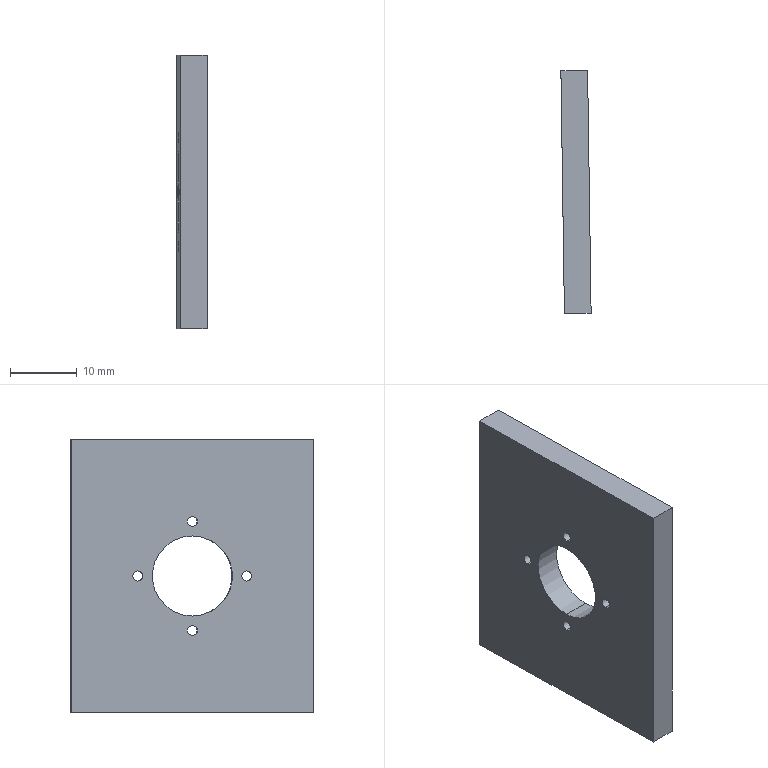Component | SolidWorks | MiddleBaffle-1 | 1 solid | 16 faces | box 4.53 x 36.32 x 41 mm | volume 5472 mm3 | cylinder 10 | plane 6 | commonest cylinder face diameters 1.5 x8 12 x2
build123d program:
from build123d import *

# Parameters (mm, degrees)
SKETCH1_2_W                 = 41
SKETCH1_2_H                 = 36.324
BOSS_EXTRUDE1_DEPTH         = 4
CUT_EXTRUDE1_DEPTH          = 56.157
CUT_EXTRUDE1_DEPTH_BACK     = 56.157
SKETCH2_R                   = 6
SKETCH3_R                   = 0.75
CUT_EXTRUDE2_DEPTH          = 56.157
CIRPATTERN1_COUNT           = 4
BOTTOM_SEAT_TRIM_DEPTH      = 56.157
BOTTOM_SEAT_TRIM_DEPTH_BACK = 56.157


with BuildPart() as part:
    # Sketch1_2 → Boss-Extrude1 (new body)
    with BuildSketch(Plane.XY):
        with Locations((1, 32.475)):
            Rectangle(SKETCH1_2_W, SKETCH1_2_H)
    extrude(amount=BOSS_EXTRUDE1_DEPTH)

    # Sketch2 → Cut-Extrude1 (cut, two sides: drawn at the far end of the back side and taken through both)
    with BuildSketch(Plane.XY.offset(4).offset(-CUT_EXTRUDE1_DEPTH_BACK)):
        with Locations((1, 32.475)):
            Circle(SKETCH2_R)
    extrude(amount=CUT_EXTRUDE1_DEPTH + CUT_EXTRUDE1_DEPTH_BACK, mode=Mode.SUBTRACT)

    # Sketch3 → Cut-Extrude2 (cut, symmetric)
    with BuildSketch(Plane.XY.offset(4)):
        with Locations((1, 40.63)):
            Circle(SKETCH3_R)
    cut_extrude2 = extrude(amount=CUT_EXTRUDE2_DEPTH, both=True, mode=Mode.SUBTRACT)

    # CirPattern1: Cut-Extrude2 ×4 about axis
    cirpattern1_axis = Axis((1, 32.475, 0), (0, 0, 1))
    for i in range(1, CIRPATTERN1_COUNT):
        add(cut_extrude2.rotate(cirpattern1_axis, i * 360 / CIRPATTERN1_COUNT), mode=Mode.SUBTRACT)

    # Sketch1 → Bottom seat trim (cut, two sides: drawn at the far end of the back side and taken through both)
    with BuildSketch(Plane(origin=(0, 0, 0), x_dir=(0, 0, -1), z_dir=(1, 0, 0)).offset(-BOTTOM_SEAT_TRIM_DEPTH_BACK)):
        Polygon((0.5, 14.305), (-4.5, 14.378), (-4.5, 13.9), (0.5, 13.9), align=None)
    extrude(amount=BOTTOM_SEAT_TRIM_DEPTH + BOTTOM_SEAT_TRIM_DEPTH_BACK, mode=Mode.SUBTRACT)


solid = part.part

# Placed as in the assembly
solid = solid.moved(Location((90.898, 1.581, 0), (90, -89.169, 90)))
STEP:
#1=COLOUR_RGB('',0.7922,0.8196,0.9333);
#2=FILL_AREA_STYLE_COLOUR('',#1);
#3=FILL_AREA_STYLE('',(#2));
#4=SURFACE_STYLE_FILL_AREA(#3);
#5=SURFACE_SIDE_STYLE('',(#4));
#6=SURFACE_STYLE_USAGE(.BOTH.,#5);
#7=PRESENTATION_STYLE_ASSIGNMENT((#6));
#8=CARTESIAN_POINT('',(3.56,1.341,-0.3112));
#9=VERTEX_POINT('',#8);
#10=CARTESIAN_POINT('',(3.56,1.341,-0.2522));
#11=VERTEX_POINT('',#10);
#12=CARTESIAN_POINT('',(3.56,1.341,-0.2817));
#13=DIRECTION('',(-0.9999,-0.0145,0.));
#14=DIRECTION('',(-0.0145,0.9999,-0.));
#15=AXIS2_PLACEMENT_3D('',#12,#13,#14);
#16=CIRCLE('',#15,0.02953);
#17=EDGE_CURVE('',#9,#11,#16,.T.);
#18=ORIENTED_EDGE('',*,*,#17,.F.);
#19=CARTESIAN_POINT('',(3.403,1.338,-0.3112));
#20=VERTEX_POINT('',#19);
#21=CARTESIAN_POINT('',(3.56,1.341,-0.3112));
#22=DIRECTION('',(-0.9999,-0.0145,0.));
#23=VECTOR('',#22,39.37);
#24=LINE('',#21,#23);
#25=EDGE_CURVE('',#9,#20,#24,.T.);
#26=ORIENTED_EDGE('',*,*,#25,.T.);
#27=CARTESIAN_POINT('',(3.403,1.338,-0.2522));
#28=VERTEX_POINT('',#27);
#29=CARTESIAN_POINT('',(3.403,1.338,-0.2817));
#30=DIRECTION('',(-0.9999,-0.0145,0.));
#31=DIRECTION('',(0.,0.,1.));
#32=AXIS2_PLACEMENT_3D('',#29,#30,#31);
#33=CIRCLE('',#32,0.02953);
#34=EDGE_CURVE('',#20,#28,#33,.T.);
#35=ORIENTED_EDGE('',*,*,#34,.T.);
#36=CARTESIAN_POINT('',(3.56,1.341,-0.2522));
#37=DIRECTION('',(-0.9999,-0.0145,0.));
#38=VECTOR('',#37,39.37);
#39=LINE('',#36,#38);
#40=EDGE_CURVE('',#11,#28,#39,.T.);
#41=ORIENTED_EDGE('',*,*,#40,.F.);
#42=EDGE_LOOP('',(#18,#26,#35,#41));
#43=FACE_OUTER_BOUND('',#42,.T.);
#44=CARTESIAN_POINT('',(3.56,1.341,-0.2817));
#45=DIRECTION('',(-0.9999,-0.0145,0.));
#46=DIRECTION('',(0.,0.,1.));
#47=AXIS2_PLACEMENT_3D('',#44,#45,#46);
#48=CYLINDRICAL_SURFACE('',#47,0.02953);
#49=ADVANCED_FACE('',(#43),#48,.F.);
#50=CARTESIAN_POINT('',(3.565,1.02,0.009843));
#51=VERTEX_POINT('',#50);
#52=CARTESIAN_POINT('',(3.565,1.02,0.0689));
#53=VERTEX_POINT('',#52);
#54=CARTESIAN_POINT('',(3.565,1.02,0.03937));
#55=DIRECTION('',(-0.9999,-0.0145,0.));
#56=DIRECTION('',(0.,0.,-1.));
#57=AXIS2_PLACEMENT_3D('',#54,#55,#56);
#58=CIRCLE('',#57,0.02953);
#59=EDGE_CURVE('',#51,#53,#58,.T.);
#60=ORIENTED_EDGE('',*,*,#59,.F.);
#61=CARTESIAN_POINT('',(3.407,1.017,0.009843));
#62=VERTEX_POINT('',#61);
#63=CARTESIAN_POINT('',(3.565,1.02,0.009843));
#64=DIRECTION('',(-0.9999,-0.0145,0.));
#65=VECTOR('',#64,39.37);
#66=LINE('',#63,#65);
#67=EDGE_CURVE('',#51,#62,#66,.T.);
#68=ORIENTED_EDGE('',*,*,#67,.T.);
#69=CARTESIAN_POINT('',(3.407,1.017,0.0689));
#70=VERTEX_POINT('',#69);
#71=CARTESIAN_POINT('',(3.407,1.017,0.03937));
#72=DIRECTION('',(-0.9999,-0.0145,0.));
#73=DIRECTION('',(0.,0.,1.));
#74=AXIS2_PLACEMENT_3D('',#71,#72,#73);
#75=CIRCLE('',#74,0.02953);
#76=EDGE_CURVE('',#62,#70,#75,.T.);
#77=ORIENTED_EDGE('',*,*,#76,.T.);
#78=CARTESIAN_POINT('',(3.565,1.02,0.0689));
#79=DIRECTION('',(-0.9999,-0.0145,0.));
#80=VECTOR('',#79,39.37);
#81=LINE('',#78,#80);
#82=EDGE_CURVE('',#53,#70,#81,.T.);
#83=ORIENTED_EDGE('',*,*,#82,.F.);
#84=EDGE_LOOP('',(#60,#68,#77,#83));
#85=FACE_OUTER_BOUND('',#84,.T.);
#86=CARTESIAN_POINT('',(3.565,1.02,0.03937));
#87=DIRECTION('',(-0.9999,-0.0145,0.));
#88=DIRECTION('',(0.,0.,1.));
#89=AXIS2_PLACEMENT_3D('',#86,#87,#88);
#90=CYLINDRICAL_SURFACE('',#89,0.02953);
#91=ADVANCED_FACE('',(#85),#90,.F.);
#92=CARTESIAN_POINT('',(3.56,1.341,0.3309));
#93=VERTEX_POINT('',#92);
#94=CARTESIAN_POINT('',(3.56,1.341,0.39));
#95=VERTEX_POINT('',#94);
#96=CARTESIAN_POINT('',(3.56,1.341,0.3604));
#97=DIRECTION('',(-0.9999,-0.0145,0.));
#98=DIRECTION('',(0.0145,-0.9999,0.));
#99=AXIS2_PLACEMENT_3D('',#96,#97,#98);
#100=CIRCLE('',#99,0.02953);
#101=EDGE_CURVE('',#93,#95,#100,.T.);
#102=ORIENTED_EDGE('',*,*,#101,.F.);
#103=CARTESIAN_POINT('',(3.403,1.338,0.3309));
#104=VERTEX_POINT('',#103);
#105=CARTESIAN_POINT('',(3.56,1.341,0.3309));
#106=DIRECTION('',(-0.9999,-0.0145,0.));
#107=VECTOR('',#106,39.37);
#108=LINE('',#105,#107);
#109=EDGE_CURVE('',#93,#104,#108,.T.);
#110=ORIENTED_EDGE('',*,*,#109,.T.);
#111=CARTESIAN_POINT('',(3.403,1.338,0.39));
#112=VERTEX_POINT('',#111);
#113=CARTESIAN_POINT('',(3.403,1.338,0.3604));
#114=DIRECTION('',(-0.9999,-0.0145,0.));
#115=DIRECTION('',(0.,0.,1.));
#116=AXIS2_PLACEMENT_3D('',#113,#114,#115);
#117=CIRCLE('',#116,0.02953);
#118=EDGE_CURVE('',#104,#112,#117,.T.);
#119=ORIENTED_EDGE('',*,*,#118,.T.);
#120=CARTESIAN_POINT('',(3.56,1.341,0.39));
#121=DIRECTION('',(-0.9999,-0.0145,0.));
#122=VECTOR('',#121,39.37);
#123=LINE('',#120,#122);
#124=EDGE_CURVE('',#95,#112,#123,.T.);
#125=ORIENTED_EDGE('',*,*,#124,.F.);
#126=EDGE_LOOP('',(#102,#110,#119,#125));
#127=FACE_OUTER_BOUND('',#126,.T.);
#128=CARTESIAN_POINT('',(3.56,1.341,0.3604));
#129=DIRECTION('',(-0.9999,-0.0145,0.));
#130=DIRECTION('',(0.,0.,1.));
#131=AXIS2_PLACEMENT_3D('',#128,#129,#130);
#132=CYLINDRICAL_SURFACE('',#131,0.02953);
#133=ADVANCED_FACE('',(#127),#132,.F.);
#134=CARTESIAN_POINT('',(3.555,1.662,0.009843));
#135=VERTEX_POINT('',#134);
#136=CARTESIAN_POINT('',(3.555,1.662,0.0689));
#137=VERTEX_POINT('',#136);
#138=CARTESIAN_POINT('',(3.555,1.662,0.03937));
#139=DIRECTION('',(-0.9999,-0.0145,0.));
#140=DIRECTION('',(0.,0.,1.));
#141=AXIS2_PLACEMENT_3D('',#138,#139,#140);
#142=CIRCLE('',#141,0.02953);
#143=EDGE_CURVE('',#135,#137,#142,.T.);
#144=ORIENTED_EDGE('',*,*,#143,.F.);
#145=CARTESIAN_POINT('',(3.398,1.659,0.009843));
#146=VERTEX_POINT('',#145);
#147=CARTESIAN_POINT('',(3.555,1.662,0.009843));
#148=DIRECTION('',(-0.9999,-0.0145,0.));
#149=VECTOR('',#148,39.37);
#150=LINE('',#147,#149);
#151=EDGE_CURVE('',#135,#146,#150,.T.);
#152=ORIENTED_EDGE('',*,*,#151,.T.);
#153=CARTESIAN_POINT('',(3.398,1.659,0.0689));
#154=VERTEX_POINT('',#153);
#155=CARTESIAN_POINT('',(3.398,1.659,0.03937));
#156=DIRECTION('',(-0.9999,-0.0145,0.));
#157=DIRECTION('',(0.,0.,1.));
#158=AXIS2_PLACEMENT_3D('',#155,#156,#157);
#159=CIRCLE('',#158,0.02953);
#160=EDGE_CURVE('',#146,#154,#159,.T.);
#161=ORIENTED_EDGE('',*,*,#160,.T.);
#162=CARTESIAN_POINT('',(3.555,1.662,0.0689));
#163=DIRECTION('',(-0.9999,-0.0145,0.));
#164=VECTOR('',#163,39.37);
#165=LINE('',#162,#164);
#166=EDGE_CURVE('',#137,#154,#165,.T.);
#167=ORIENTED_EDGE('',*,*,#166,.F.);
#168=EDGE_LOOP('',(#144,#152,#161,#167));
#169=FACE_OUTER_BOUND('',#168,.T.);
#170=CARTESIAN_POINT('',(3.555,1.662,0.03937));
#171=DIRECTION('',(-0.9999,-0.0145,0.));
#172=DIRECTION('',(0.,0.,1.));
#173=AXIS2_PLACEMENT_3D('',#170,#171,#172);
#174=CYLINDRICAL_SURFACE('',#173,0.02953);
#175=ADVANCED_FACE('',(#169),#174,.F.);
#176=CARTESIAN_POINT('',(3.56,1.341,-0.1969));
#177=VERTEX_POINT('',#176);
#178=CARTESIAN_POINT('',(3.56,1.341,0.2756));
#179=VERTEX_POINT('',#178);
#180=CARTESIAN_POINT('',(3.56,1.341,0.03937));
#181=DIRECTION('',(-0.9999,-0.0145,0.));
#182=DIRECTION('',(0.,0.,1.));
#183=AXIS2_PLACEMENT_3D('',#180,#181,#182);
#184=CIRCLE('',#183,0.2362);
#185=EDGE_CURVE('',#177,#179,#184,.T.);
#186=ORIENTED_EDGE('',*,*,#185,.F.);
#187=CARTESIAN_POINT('',(3.403,1.338,-0.1969));
#188=VERTEX_POINT('',#187);
#189=CARTESIAN_POINT('',(3.56,1.341,-0.1969));
#190=DIRECTION('',(-0.9999,-0.0145,0.));
#191=VECTOR('',#190,39.37);
#192=LINE('',#189,#191);
#193=EDGE_CURVE('',#177,#188,#192,.T.);
#194=ORIENTED_EDGE('',*,*,#193,.T.);
#195=CARTESIAN_POINT('',(3.403,1.338,0.2756));
#196=VERTEX_POINT('',#195);
#197=CARTESIAN_POINT('',(3.403,1.338,0.03937));
#198=DIRECTION('',(-0.9999,-0.0145,0.));
#199=DIRECTION('',(0.,0.,1.));
#200=AXIS2_PLACEMENT_3D('',#197,#198,#199);
#201=CIRCLE('',#200,0.2362);
#202=EDGE_CURVE('',#188,#196,#201,.T.);
#203=ORIENTED_EDGE('',*,*,#202,.T.);
#204=CARTESIAN_POINT('',(3.56,1.341,0.2756));
#205=DIRECTION('',(-0.9999,-0.0145,0.));
#206=VECTOR('',#205,39.37);
#207=LINE('',#204,#206);
#208=EDGE_CURVE('',#179,#196,#207,.T.);
#209=ORIENTED_EDGE('',*,*,#208,.F.);
#210=EDGE_LOOP('',(#186,#194,#203,#209));
#211=FACE_OUTER_BOUND('',#210,.T.);
#212=CARTESIAN_POINT('',(3.56,1.341,0.03937));
#213=DIRECTION('',(-0.9999,-0.0145,0.));
#214=DIRECTION('',(0.,0.,1.));
#215=AXIS2_PLACEMENT_3D('',#212,#213,#214);
#216=CYLINDRICAL_SURFACE('',#215,0.2362);
#217=ADVANCED_FACE('',(#211),#216,.F.);
#218=CARTESIAN_POINT('',(3.57,0.6257,0.8465));
#219=VERTEX_POINT('',#218);
#220=CARTESIAN_POINT('',(3.413,0.6257,0.8465));
#221=VERTEX_POINT('',#220);
#222=CARTESIAN_POINT('',(3.59,0.6257,0.8465));
#223=DIRECTION('',(-1.,0.0000005,0.));
#224=VECTOR('',#223,39.37);
#225=LINE('',#222,#224);
#226=EDGE_CURVE('',#219,#221,#225,.T.);
#227=ORIENTED_EDGE('',*,*,#226,.F.);
#228=CARTESIAN_POINT('',(3.55,2.056,0.8465));
#229=VERTEX_POINT('',#228);
#230=CARTESIAN_POINT('',(3.55,2.056,0.8465));
#231=DIRECTION('',(-0.0145,0.9999,0.));
#232=VECTOR('',#231,39.37);
#233=LINE('',#230,#232);
#234=EDGE_CURVE('',#219,#229,#233,.T.);
#235=ORIENTED_EDGE('',*,*,#234,.T.);
#236=CARTESIAN_POINT('',(3.392,2.053,0.8465));
#237=VERTEX_POINT('',#236);
#238=CARTESIAN_POINT('',(3.392,2.053,0.8465));
#239=DIRECTION('',(0.9999,0.0145,0.));
#240=VECTOR('',#239,39.37);
#241=LINE('',#238,#240);
#242=EDGE_CURVE('',#237,#229,#241,.T.);
#243=ORIENTED_EDGE('',*,*,#242,.F.);
#244=CARTESIAN_POINT('',(3.392,2.053,0.8465));
#245=DIRECTION('',(-0.0145,0.9999,0.));
#246=VECTOR('',#245,39.37);
#247=LINE('',#244,#246);
#248=EDGE_CURVE('',#221,#237,#247,.T.);
#249=ORIENTED_EDGE('',*,*,#248,.F.);
#250=EDGE_LOOP('',(#227,#235,#243,#249));
#251=FACE_OUTER_BOUND('',#250,.T.);
#252=CARTESIAN_POINT('',(3.392,2.053,0.8465));
#253=DIRECTION('',(0.,0.,-1.));
#254=DIRECTION('',(-0.9999,-0.0145,0.));
#255=AXIS2_PLACEMENT_3D('',#252,#253,#254);
#256=PLANE('',#255);
#257=ADVANCED_FACE('',(#251),#256,.F.);
#258=CARTESIAN_POINT('',(3.55,2.056,-0.7677));
#259=VERTEX_POINT('',#258);
#260=CARTESIAN_POINT('',(3.57,0.6257,-0.7677));
#261=VERTEX_POINT('',#260);
#262=CARTESIAN_POINT('',(3.55,2.056,-0.7677));
#263=DIRECTION('',(0.0145,-0.9999,0.));
#264=VECTOR('',#263,39.37);
#265=LINE('',#262,#264);
#266=EDGE_CURVE('',#259,#261,#265,.T.);
#267=ORIENTED_EDGE('',*,*,#266,.T.);
#268=CARTESIAN_POINT('',(3.413,0.6257,-0.7677));
#269=VERTEX_POINT('',#268);
#270=CARTESIAN_POINT('',(3.59,0.6257,-0.7677));
#271=DIRECTION('',(-1.,0.0000005,0.));
#272=VECTOR('',#271,39.37);
#273=LINE('',#270,#272);
#274=EDGE_CURVE('',#261,#269,#273,.T.);
#275=ORIENTED_EDGE('',*,*,#274,.T.);
#276=CARTESIAN_POINT('',(3.392,2.053,-0.7677));
#277=VERTEX_POINT('',#276);
#278=CARTESIAN_POINT('',(3.392,2.053,-0.7677));
#279=DIRECTION('',(0.0145,-0.9999,0.));
#280=VECTOR('',#279,39.37);
#281=LINE('',#278,#280);
#282=EDGE_CURVE('',#277,#269,#281,.T.);
#283=ORIENTED_EDGE('',*,*,#282,.F.);
#284=CARTESIAN_POINT('',(3.392,2.053,-0.7677));
#285=DIRECTION('',(0.9999,0.0145,0.));
#286=VECTOR('',#285,39.37);
#287=LINE('',#284,#286);
#288=EDGE_CURVE('',#277,#259,#287,.T.);
#289=ORIENTED_EDGE('',*,*,#288,.T.);
#290=EDGE_LOOP('',(#267,#275,#283,#289));
#291=FACE_OUTER_BOUND('',#290,.T.);
#292=CARTESIAN_POINT('',(3.392,2.053,-0.7677));
#293=DIRECTION('',(0.,0.,1.));
#294=DIRECTION('',(0.9999,0.0145,0.));
#295=AXIS2_PLACEMENT_3D('',#292,#293,#294);
#296=PLANE('',#295);
#297=ADVANCED_FACE('',(#291),#296,.F.);
#298=CARTESIAN_POINT('',(3.55,2.056,-0.7677));
#299=DIRECTION('',(0.,0.,-1.));
#300=VECTOR('',#299,39.37);
#301=LINE('',#298,#300);
#302=EDGE_CURVE('',#229,#259,#301,.T.);
#303=ORIENTED_EDGE('',*,*,#302,.T.);
#304=ORIENTED_EDGE('',*,*,#288,.F.);
#305=CARTESIAN_POINT('',(3.392,2.053,-0.7677));
#306=DIRECTION('',(0.,0.,-1.));
#307=VECTOR('',#306,39.37);
#308=LINE('',#305,#307);
#309=EDGE_CURVE('',#237,#277,#308,.T.);
#310=ORIENTED_EDGE('',*,*,#309,.F.);
#311=ORIENTED_EDGE('',*,*,#242,.T.);
#312=EDGE_LOOP('',(#303,#304,#310,#311));
#313=FACE_OUTER_BOUND('',#312,.T.);
#314=CARTESIAN_POINT('',(3.392,2.053,-0.7677));
#315=DIRECTION('',(0.0145,-0.9999,0.));
#316=DIRECTION('',(0.9999,0.0145,0.));
#317=AXIS2_PLACEMENT_3D('',#314,#315,#316);
#318=PLANE('',#317);
#319=ADVANCED_FACE('',(#313),#318,.F.);
#320=CARTESIAN_POINT('',(3.413,0.6257,0.));
#321=DIRECTION('',(0.,0.,-1.));
#322=VECTOR('',#321,39.37);
#323=LINE('',#320,#322);
#324=EDGE_CURVE('',#221,#269,#323,.T.);
#325=ORIENTED_EDGE('',*,*,#324,.F.);
#326=ORIENTED_EDGE('',*,*,#248,.T.);
#327=ORIENTED_EDGE('',*,*,#309,.T.);
#328=ORIENTED_EDGE('',*,*,#282,.T.);
#329=EDGE_LOOP('',(#325,#326,#327,#328));
#330=FACE_OUTER_BOUND('',#329,.T.);
#331=CARTESIAN_POINT('',(3.403,1.338,-0.2817));
#332=DIRECTION('',(-0.9999,-0.0145,0.));
#333=DIRECTION('',(0.,0.,1.));
#334=AXIS2_PLACEMENT_3D('',#331,#332,#333);
#335=CIRCLE('',#334,0.02953);
#336=EDGE_CURVE('',#28,#20,#335,.T.);
#337=ORIENTED_EDGE('',*,*,#336,.F.);
#338=ORIENTED_EDGE('',*,*,#34,.F.);
#339=EDGE_LOOP('',(#337,#338));
#340=FACE_BOUND('',#339,.T.);
#341=CARTESIAN_POINT('',(3.407,1.017,0.03937));
#342=DIRECTION('',(-0.9999,-0.0145,0.));
#343=DIRECTION('',(0.,0.,1.));
#344=AXIS2_PLACEMENT_3D('',#341,#342,#343);
#345=CIRCLE('',#344,0.02953);
#346=EDGE_CURVE('',#70,#62,#345,.T.);
#347=ORIENTED_EDGE('',*,*,#346,.F.);
#348=ORIENTED_EDGE('',*,*,#76,.F.);
#349=EDGE_LOOP('',(#347,#348));
#350=FACE_BOUND('',#349,.T.);
#351=CARTESIAN_POINT('',(3.403,1.338,0.3604));
#352=DIRECTION('',(-0.9999,-0.0145,0.));
#353=DIRECTION('',(0.,0.,1.));
#354=AXIS2_PLACEMENT_3D('',#351,#352,#353);
#355=CIRCLE('',#354,0.02953);
#356=EDGE_CURVE('',#112,#104,#355,.T.);
#357=ORIENTED_EDGE('',*,*,#356,.F.);
#358=ORIENTED_EDGE('',*,*,#118,.F.);
#359=EDGE_LOOP('',(#357,#358));
#360=FACE_BOUND('',#359,.T.);
#361=CARTESIAN_POINT('',(3.398,1.659,0.03937));
#362=DIRECTION('',(-0.9999,-0.0145,0.));
#363=DIRECTION('',(0.,0.,1.));
#364=AXIS2_PLACEMENT_3D('',#361,#362,#363);
#365=CIRCLE('',#364,0.02953);
#366=EDGE_CURVE('',#154,#146,#365,.T.);
#367=ORIENTED_EDGE('',*,*,#366,.F.);
#368=ORIENTED_EDGE('',*,*,#160,.F.);
#369=EDGE_LOOP('',(#367,#368));
#370=FACE_BOUND('',#369,.T.);
#371=CARTESIAN_POINT('',(3.403,1.338,0.03937));
#372=DIRECTION('',(-0.9999,-0.0145,0.));
#373=DIRECTION('',(0.,0.,1.));
#374=AXIS2_PLACEMENT_3D('',#371,#372,#373);
#375=CIRCLE('',#374,0.2362);
#376=EDGE_CURVE('',#196,#188,#375,.T.);
#377=ORIENTED_EDGE('',*,*,#376,.F.);
#378=ORIENTED_EDGE('',*,*,#202,.F.);
#379=EDGE_LOOP('',(#377,#378));
#380=FACE_BOUND('',#379,.T.);
#381=CARTESIAN_POINT('',(3.421,0.05994,0.));
#382=DIRECTION('',(-0.9999,-0.0145,0.));
#383=DIRECTION('',(0.,0.,1.));
#384=AXIS2_PLACEMENT_3D('',#381,#382,#383);
#385=PLANE('',#384);
#386=ADVANCED_FACE('',(#330,#340,#350,#360,#370,#380),#385,.T.);
#387=CARTESIAN_POINT('',(3.56,1.341,-0.2817));
#388=DIRECTION('',(-0.9999,-0.0145,0.));
#389=DIRECTION('',(-0.0145,0.9999,-0.));
#390=AXIS2_PLACEMENT_3D('',#387,#388,#389);
#391=CIRCLE('',#390,0.02953);
#392=EDGE_CURVE('',#11,#9,#391,.T.);
#393=ORIENTED_EDGE('',*,*,#392,.T.);
#394=ORIENTED_EDGE('',*,*,#17,.T.);
#395=EDGE_LOOP('',(#393,#394));
#396=FACE_BOUND('',#395,.T.);
#397=CARTESIAN_POINT('',(3.565,1.02,0.03937));
#398=DIRECTION('',(-0.9999,-0.0145,0.));
#399=DIRECTION('',(0.,0.,-1.));
#400=AXIS2_PLACEMENT_3D('',#397,#398,#399);
#401=CIRCLE('',#400,0.02953);
#402=EDGE_CURVE('',#53,#51,#401,.T.);
#403=ORIENTED_EDGE('',*,*,#402,.T.);
#404=ORIENTED_EDGE('',*,*,#59,.T.);
#405=EDGE_LOOP('',(#403,#404));
#406=FACE_BOUND('',#405,.T.);
#407=CARTESIAN_POINT('',(3.56,1.341,0.3604));
#408=DIRECTION('',(-0.9999,-0.0145,0.));
#409=DIRECTION('',(0.0145,-0.9999,0.));
#410=AXIS2_PLACEMENT_3D('',#407,#408,#409);
#411=CIRCLE('',#410,0.02953);
#412=EDGE_CURVE('',#95,#93,#411,.T.);
#413=ORIENTED_EDGE('',*,*,#412,.T.);
#414=ORIENTED_EDGE('',*,*,#101,.T.);
#415=EDGE_LOOP('',(#413,#414));
#416=FACE_BOUND('',#415,.T.);
#417=CARTESIAN_POINT('',(3.555,1.662,0.03937));
#418=DIRECTION('',(-0.9999,-0.0145,0.));
#419=DIRECTION('',(0.,0.,1.));
#420=AXIS2_PLACEMENT_3D('',#417,#418,#419);
#421=CIRCLE('',#420,0.02953);
#422=EDGE_CURVE('',#137,#135,#421,.T.);
#423=ORIENTED_EDGE('',*,*,#422,.T.);
#424=ORIENTED_EDGE('',*,*,#143,.T.);
#425=EDGE_LOOP('',(#423,#424));
#426=FACE_BOUND('',#425,.T.);
#427=CARTESIAN_POINT('',(3.56,1.341,0.03937));
#428=DIRECTION('',(-0.9999,-0.0145,0.));
#429=DIRECTION('',(0.,0.,1.));
#430=AXIS2_PLACEMENT_3D('',#427,#428,#429);
#431=CIRCLE('',#430,0.2362);
#432=EDGE_CURVE('',#179,#177,#431,.T.);
#433=ORIENTED_EDGE('',*,*,#432,.T.);
#434=ORIENTED_EDGE('',*,*,#185,.T.);
#435=EDGE_LOOP('',(#433,#434));
#436=FACE_BOUND('',#435,.T.);
#437=ORIENTED_EDGE('',*,*,#234,.F.);
#438=CARTESIAN_POINT('',(3.57,0.6257,0.));
#439=DIRECTION('',(0.,0.,-1.));
#440=VECTOR('',#439,39.37);
#441=LINE('',#438,#440);
#442=EDGE_CURVE('',#219,#261,#441,.T.);
#443=ORIENTED_EDGE('',*,*,#442,.T.);
#444=ORIENTED_EDGE('',*,*,#266,.F.);
#445=ORIENTED_EDGE('',*,*,#302,.F.);
#446=EDGE_LOOP('',(#437,#443,#444,#445));
#447=FACE_OUTER_BOUND('',#446,.T.);
#448=CARTESIAN_POINT('',(3.579,0.06223,0.));
#449=DIRECTION('',(-0.9999,-0.0145,0.));
#450=DIRECTION('',(0.,0.,1.));
#451=AXIS2_PLACEMENT_3D('',#448,#449,#450);
#452=PLANE('',#451);
#453=ADVANCED_FACE('',(#396,#406,#416,#426,#436,#447),#452,.F.);
#454=ORIENTED_EDGE('',*,*,#193,.F.);
#455=ORIENTED_EDGE('',*,*,#432,.F.);
#456=ORIENTED_EDGE('',*,*,#208,.T.);
#457=ORIENTED_EDGE('',*,*,#376,.T.);
#458=EDGE_LOOP('',(#454,#455,#456,#457));
#459=FACE_OUTER_BOUND('',#458,.T.);
#460=CARTESIAN_POINT('',(3.56,1.341,0.03937));
#461=DIRECTION('',(-0.9999,-0.0145,0.));
#462=DIRECTION('',(0.,0.,1.));
#463=AXIS2_PLACEMENT_3D('',#460,#461,#462);
#464=CYLINDRICAL_SURFACE('',#463,0.2362);
#465=ADVANCED_FACE('',(#459),#464,.F.);
#466=ORIENTED_EDGE('',*,*,#151,.F.);
#467=ORIENTED_EDGE('',*,*,#422,.F.);
#468=ORIENTED_EDGE('',*,*,#166,.T.);
#469=ORIENTED_EDGE('',*,*,#366,.T.);
#470=EDGE_LOOP('',(#466,#467,#468,#469));
#471=FACE_OUTER_BOUND('',#470,.T.);
#472=CARTESIAN_POINT('',(3.555,1.662,0.03937));
#473=DIRECTION('',(-0.9999,-0.0145,0.));
#474=DIRECTION('',(0.,0.,1.));
#475=AXIS2_PLACEMENT_3D('',#472,#473,#474);
#476=CYLINDRICAL_SURFACE('',#475,0.02953);
#477=ADVANCED_FACE('',(#471),#476,.F.);
#478=ORIENTED_EDGE('',*,*,#109,.F.);
#479=ORIENTED_EDGE('',*,*,#412,.F.);
#480=ORIENTED_EDGE('',*,*,#124,.T.);
#481=ORIENTED_EDGE('',*,*,#356,.T.);
#482=EDGE_LOOP('',(#478,#479,#480,#481));
#483=FACE_OUTER_BOUND('',#482,.T.);
#484=CARTESIAN_POINT('',(3.56,1.341,0.3604));
#485=DIRECTION('',(-0.9999,-0.0145,0.));
#486=DIRECTION('',(0.,0.,1.));
#487=AXIS2_PLACEMENT_3D('',#484,#485,#486);
#488=CYLINDRICAL_SURFACE('',#487,0.02953);
#489=ADVANCED_FACE('',(#483),#488,.F.);
#490=ORIENTED_EDGE('',*,*,#67,.F.);
#491=ORIENTED_EDGE('',*,*,#402,.F.);
#492=ORIENTED_EDGE('',*,*,#82,.T.);
#493=ORIENTED_EDGE('',*,*,#346,.T.);
#494=EDGE_LOOP('',(#490,#491,#492,#493));
#495=FACE_OUTER_BOUND('',#494,.T.);
#496=CARTESIAN_POINT('',(3.565,1.02,0.03937));
#497=DIRECTION('',(-0.9999,-0.0145,0.));
#498=DIRECTION('',(0.,0.,1.));
#499=AXIS2_PLACEMENT_3D('',#496,#497,#498);
#500=CYLINDRICAL_SURFACE('',#499,0.02953);
#501=ADVANCED_FACE('',(#495),#500,.F.);
#502=ORIENTED_EDGE('',*,*,#25,.F.);
#503=ORIENTED_EDGE('',*,*,#392,.F.);
#504=ORIENTED_EDGE('',*,*,#40,.T.);
#505=ORIENTED_EDGE('',*,*,#336,.T.);
#506=EDGE_LOOP('',(#502,#503,#504,#505));
#507=FACE_OUTER_BOUND('',#506,.T.);
#508=CARTESIAN_POINT('',(3.56,1.341,-0.2817));
#509=DIRECTION('',(-0.9999,-0.0145,0.));
#510=DIRECTION('',(0.,0.,1.));
#511=AXIS2_PLACEMENT_3D('',#508,#509,#510);
#512=CYLINDRICAL_SURFACE('',#511,0.02953);
#513=ADVANCED_FACE('',(#507),#512,.F.);
#514=ORIENTED_EDGE('',*,*,#324,.T.);
#515=ORIENTED_EDGE('',*,*,#274,.F.);
#516=ORIENTED_EDGE('',*,*,#442,.F.);
#517=ORIENTED_EDGE('',*,*,#226,.T.);
#518=EDGE_LOOP('',(#514,#515,#516,#517));
#519=FACE_OUTER_BOUND('',#518,.T.);
#520=CARTESIAN_POINT('',(3.59,0.6257,-0.7677));
#521=DIRECTION('',(0.0000005,1.,0.));
#522=DIRECTION('',(-1.,0.0000005,0.));
#523=AXIS2_PLACEMENT_3D('',#520,#521,#522);
#524=PLANE('',#523);
#525=ADVANCED_FACE('',(#519),#524,.F.);
#526=CLOSED_SHELL('',(#49,#91,#133,#175,#217,#257,#297,#319,#386,#453,#465,#477,#489,#501,#513,#525));
#527=MANIFOLD_SOLID_BREP('',#526);
#528=STYLED_ITEM('',(#7),#527);
#529=PRESENTATION_LAYER_ASSIGNMENT('','',(#528));
#530=(LENGTH_UNIT()NAMED_UNIT(*)SI_UNIT($,.METRE.));
#531=LENGTH_MEASURE_WITH_UNIT(LENGTH_MEASURE(0.0254),#530);
#532=DIMENSIONAL_EXPONENTS(1.,0.,0.,0.,0.,0.,0.);
#533=(CONVERSION_BASED_UNIT('',#531)LENGTH_UNIT()NAMED_UNIT(#532));
#534=UNCERTAINTY_MEASURE_WITH_UNIT(LENGTH_MEASURE(0.00001),#533,'','');
#535=(NAMED_UNIT(*)PLANE_ANGLE_UNIT()SI_UNIT($,.RADIAN.));
#536=(NAMED_UNIT(*)SI_UNIT($,.STERADIAN.)SOLID_ANGLE_UNIT());
#537=(GEOMETRIC_REPRESENTATION_CONTEXT(3)GLOBAL_UNCERTAINTY_ASSIGNED_CONTEXT((#534))GLOBAL_UNIT_ASSIGNED_CONTEXT((#533,#535,#536))REPRESENTATION_CONTEXT('',''));
#538=MECHANICAL_DESIGN_GEOMETRIC_PRESENTATION_REPRESENTATION('',(#528),#537);
#539=CARTESIAN_POINT('',(0.,0.,0.));
#540=DIRECTION('',(0.,0.,1.));
#541=DIRECTION('',(1.,0.,0.));
#542=AXIS2_PLACEMENT_3D('',#539,#540,#541);
#543=(LENGTH_UNIT()NAMED_UNIT(*)SI_UNIT($,.METRE.));
#544=LENGTH_MEASURE_WITH_UNIT(LENGTH_MEASURE(0.0254),#543);
#545=DIMENSIONAL_EXPONENTS(1.,0.,0.,0.,0.,0.,0.);
#546=(CONVERSION_BASED_UNIT('',#544)LENGTH_UNIT()NAMED_UNIT(#545));
#547=UNCERTAINTY_MEASURE_WITH_UNIT(LENGTH_MEASURE(0.00001),#546,'','');
#548=(NAMED_UNIT(*)PLANE_ANGLE_UNIT()SI_UNIT($,.RADIAN.));
#549=(NAMED_UNIT(*)SI_UNIT($,.STERADIAN.)SOLID_ANGLE_UNIT());
#550=(GEOMETRIC_REPRESENTATION_CONTEXT(3)GLOBAL_UNCERTAINTY_ASSIGNED_CONTEXT((#547))GLOBAL_UNIT_ASSIGNED_CONTEXT((#546,#548,#549))REPRESENTATION_CONTEXT('',''));
#551=ADVANCED_BREP_SHAPE_REPRESENTATION('',(#527,#542),#550);